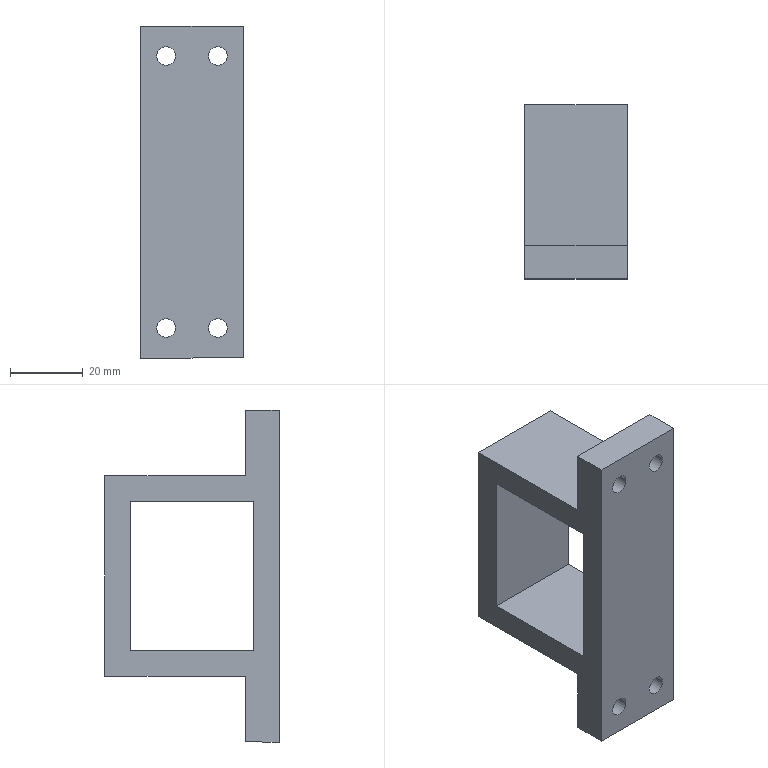Component | SolidWorks | EndCap-2 | 1 solid | 22 faces | box 28 x 47.79 x 91 mm | volume 43383 mm3 | plane 14 | cylinder 8 | commonest cylinder face diameters 5.084 x8
STEP:
#1=CARTESIAN_POINT('',(6.308,1.43,1.468));
#2=VERTEX_POINT('',#1);
#3=CARTESIAN_POINT('',(6.108,1.43,1.468));
#4=VERTEX_POINT('',#3);
#5=CARTESIAN_POINT('',(6.208,1.43,1.468));
#6=DIRECTION('',(0.,-1.,-0.));
#7=DIRECTION('',(0.,0.,-1.));
#8=AXIS2_PLACEMENT_3D('',#5,#6,#7);
#9=CIRCLE('',#8,0.1001);
#10=EDGE_CURVE('',#2,#4,#9,.T.);
#11=ORIENTED_EDGE('',*,*,#10,.T.);
#12=CARTESIAN_POINT('',(6.108,1.794,1.468));
#13=VERTEX_POINT('',#12);
#14=CARTESIAN_POINT('',(6.108,1.263,1.468));
#15=DIRECTION('',(-0.,1.,0.));
#16=VECTOR('',#15,39.37);
#17=LINE('',#14,#16);
#18=EDGE_CURVE('',#4,#13,#17,.T.);
#19=ORIENTED_EDGE('',*,*,#18,.T.);
#20=CARTESIAN_POINT('',(6.308,1.794,1.468));
#21=VERTEX_POINT('',#20);
#22=CARTESIAN_POINT('',(6.208,1.794,1.468));
#23=DIRECTION('',(-0.,1.,0.));
#24=DIRECTION('',(-1.,0.,0.));
#25=AXIS2_PLACEMENT_3D('',#22,#23,#24);
#26=CIRCLE('',#25,0.1001);
#27=EDGE_CURVE('',#13,#21,#26,.T.);
#28=ORIENTED_EDGE('',*,*,#27,.T.);
#29=CARTESIAN_POINT('',(6.308,1.263,1.468));
#30=DIRECTION('',(-0.,1.,0.));
#31=VECTOR('',#30,39.37);
#32=LINE('',#29,#31);
#33=EDGE_CURVE('',#2,#21,#32,.T.);
#34=ORIENTED_EDGE('',*,*,#33,.F.);
#35=EDGE_LOOP('',(#11,#19,#28,#34));
#36=FACE_OUTER_BOUND('',#35,.T.);
#37=CARTESIAN_POINT('',(6.208,1.263,1.468));
#38=DIRECTION('',(-0.,1.,0.));
#39=DIRECTION('',(1.,0.,0.));
#40=AXIS2_PLACEMENT_3D('',#37,#38,#39);
#41=CYLINDRICAL_SURFACE('',#40,0.1001);
#42=ADVANCED_FACE('',(#36),#41,.F.);
#43=CARTESIAN_POINT('',(6.867,1.43,1.468));
#44=VERTEX_POINT('',#43);
#45=CARTESIAN_POINT('',(6.667,1.43,1.468));
#46=VERTEX_POINT('',#45);
#47=CARTESIAN_POINT('',(6.767,1.43,1.468));
#48=DIRECTION('',(0.,-1.,-0.));
#49=DIRECTION('',(0.,0.,-1.));
#50=AXIS2_PLACEMENT_3D('',#47,#48,#49);
#51=CIRCLE('',#50,0.1001);
#52=EDGE_CURVE('',#44,#46,#51,.T.);
#53=ORIENTED_EDGE('',*,*,#52,.T.);
#54=CARTESIAN_POINT('',(6.667,1.794,1.468));
#55=VERTEX_POINT('',#54);
#56=CARTESIAN_POINT('',(6.667,1.263,1.468));
#57=DIRECTION('',(-0.,1.,0.));
#58=VECTOR('',#57,39.37);
#59=LINE('',#56,#58);
#60=EDGE_CURVE('',#46,#55,#59,.T.);
#61=ORIENTED_EDGE('',*,*,#60,.T.);
#62=CARTESIAN_POINT('',(6.867,1.794,1.468));
#63=VERTEX_POINT('',#62);
#64=CARTESIAN_POINT('',(6.767,1.794,1.468));
#65=DIRECTION('',(-0.,1.,0.));
#66=DIRECTION('',(1.,0.,0.));
#67=AXIS2_PLACEMENT_3D('',#64,#65,#66);
#68=CIRCLE('',#67,0.1001);
#69=EDGE_CURVE('',#55,#63,#68,.T.);
#70=ORIENTED_EDGE('',*,*,#69,.T.);
#71=CARTESIAN_POINT('',(6.867,1.263,1.468));
#72=DIRECTION('',(-0.,1.,0.));
#73=VECTOR('',#72,39.37);
#74=LINE('',#71,#73);
#75=EDGE_CURVE('',#44,#63,#74,.T.);
#76=ORIENTED_EDGE('',*,*,#75,.F.);
#77=EDGE_LOOP('',(#53,#61,#70,#76));
#78=FACE_OUTER_BOUND('',#77,.T.);
#79=CARTESIAN_POINT('',(6.767,1.263,1.468));
#80=DIRECTION('',(-0.,1.,0.));
#81=DIRECTION('',(1.,0.,0.));
#82=AXIS2_PLACEMENT_3D('',#79,#80,#81);
#83=CYLINDRICAL_SURFACE('',#82,0.1001);
#84=ADVANCED_FACE('',(#78),#83,.F.);
#85=CARTESIAN_POINT('',(6.867,1.43,-1.468));
#86=VERTEX_POINT('',#85);
#87=CARTESIAN_POINT('',(6.667,1.43,-1.468));
#88=VERTEX_POINT('',#87);
#89=CARTESIAN_POINT('',(6.767,1.43,-1.468));
#90=DIRECTION('',(0.,-1.,-0.));
#91=DIRECTION('',(0.,0.,-1.));
#92=AXIS2_PLACEMENT_3D('',#89,#90,#91);
#93=CIRCLE('',#92,0.1001);
#94=EDGE_CURVE('',#86,#88,#93,.T.);
#95=ORIENTED_EDGE('',*,*,#94,.T.);
#96=CARTESIAN_POINT('',(6.667,1.794,-1.468));
#97=VERTEX_POINT('',#96);
#98=CARTESIAN_POINT('',(6.667,1.263,-1.468));
#99=DIRECTION('',(-0.,1.,0.));
#100=VECTOR('',#99,39.37);
#101=LINE('',#98,#100);
#102=EDGE_CURVE('',#88,#97,#101,.T.);
#103=ORIENTED_EDGE('',*,*,#102,.T.);
#104=CARTESIAN_POINT('',(6.867,1.794,-1.468));
#105=VERTEX_POINT('',#104);
#106=CARTESIAN_POINT('',(6.767,1.794,-1.468));
#107=DIRECTION('',(-0.,1.,0.));
#108=DIRECTION('',(-1.,0.,0.));
#109=AXIS2_PLACEMENT_3D('',#106,#107,#108);
#110=CIRCLE('',#109,0.1001);
#111=EDGE_CURVE('',#97,#105,#110,.T.);
#112=ORIENTED_EDGE('',*,*,#111,.T.);
#113=CARTESIAN_POINT('',(6.867,1.263,-1.468));
#114=DIRECTION('',(-0.,1.,0.));
#115=VECTOR('',#114,39.37);
#116=LINE('',#113,#115);
#117=EDGE_CURVE('',#86,#105,#116,.T.);
#118=ORIENTED_EDGE('',*,*,#117,.F.);
#119=EDGE_LOOP('',(#95,#103,#112,#118));
#120=FACE_OUTER_BOUND('',#119,.T.);
#121=CARTESIAN_POINT('',(6.767,1.263,-1.468));
#122=DIRECTION('',(-0.,1.,0.));
#123=DIRECTION('',(1.,0.,0.));
#124=AXIS2_PLACEMENT_3D('',#121,#122,#123);
#125=CYLINDRICAL_SURFACE('',#124,0.1001);
#126=ADVANCED_FACE('',(#120),#125,.F.);
#127=CARTESIAN_POINT('',(6.308,1.43,-1.468));
#128=VERTEX_POINT('',#127);
#129=CARTESIAN_POINT('',(6.108,1.43,-1.468));
#130=VERTEX_POINT('',#129);
#131=CARTESIAN_POINT('',(6.208,1.43,-1.468));
#132=DIRECTION('',(0.,-1.,-0.));
#133=DIRECTION('',(0.,0.,-1.));
#134=AXIS2_PLACEMENT_3D('',#131,#132,#133);
#135=CIRCLE('',#134,0.1001);
#136=EDGE_CURVE('',#128,#130,#135,.T.);
#137=ORIENTED_EDGE('',*,*,#136,.T.);
#138=CARTESIAN_POINT('',(6.108,1.794,-1.468));
#139=VERTEX_POINT('',#138);
#140=CARTESIAN_POINT('',(6.108,1.263,-1.468));
#141=DIRECTION('',(-0.,1.,0.));
#142=VECTOR('',#141,39.37);
#143=LINE('',#140,#142);
#144=EDGE_CURVE('',#130,#139,#143,.T.);
#145=ORIENTED_EDGE('',*,*,#144,.T.);
#146=CARTESIAN_POINT('',(6.308,1.794,-1.468));
#147=VERTEX_POINT('',#146);
#148=CARTESIAN_POINT('',(6.208,1.794,-1.468));
#149=DIRECTION('',(-0.,1.,0.));
#150=DIRECTION('',(1.,0.,0.));
#151=AXIS2_PLACEMENT_3D('',#148,#149,#150);
#152=CIRCLE('',#151,0.1001);
#153=EDGE_CURVE('',#139,#147,#152,.T.);
#154=ORIENTED_EDGE('',*,*,#153,.T.);
#155=CARTESIAN_POINT('',(6.308,1.263,-1.468));
#156=DIRECTION('',(-0.,1.,0.));
#157=VECTOR('',#156,39.37);
#158=LINE('',#155,#157);
#159=EDGE_CURVE('',#128,#147,#158,.T.);
#160=ORIENTED_EDGE('',*,*,#159,.F.);
#161=EDGE_LOOP('',(#137,#145,#154,#160));
#162=FACE_OUTER_BOUND('',#161,.T.);
#163=CARTESIAN_POINT('',(6.208,1.263,-1.468));
#164=DIRECTION('',(-0.,1.,0.));
#165=DIRECTION('',(1.,0.,0.));
#166=AXIS2_PLACEMENT_3D('',#163,#164,#165);
#167=CYLINDRICAL_SURFACE('',#166,0.1001);
#168=ADVANCED_FACE('',(#162),#167,.F.);
#169=CARTESIAN_POINT('',(5.936,3.312,1.083));
#170=VERTEX_POINT('',#169);
#171=CARTESIAN_POINT('',(7.039,3.312,1.083));
#172=VERTEX_POINT('',#171);
#173=CARTESIAN_POINT('',(6.251,3.312,1.083));
#174=DIRECTION('',(1.,0.,0.));
#175=VECTOR('',#174,39.37);
#176=LINE('',#173,#175);
#177=EDGE_CURVE('',#170,#172,#176,.T.);
#178=ORIENTED_EDGE('',*,*,#177,.F.);
#179=CARTESIAN_POINT('',(5.936,1.794,1.083));
#180=VERTEX_POINT('',#179);
#181=CARTESIAN_POINT('',(5.936,1.794,1.083));
#182=DIRECTION('',(0.,-1.,-0.));
#183=VECTOR('',#182,39.37);
#184=LINE('',#181,#183);
#185=EDGE_CURVE('',#170,#180,#184,.T.);
#186=ORIENTED_EDGE('',*,*,#185,.T.);
#187=CARTESIAN_POINT('',(7.039,1.794,1.083));
#188=VERTEX_POINT('',#187);
#189=CARTESIAN_POINT('',(-3.832,1.794,1.083));
#190=DIRECTION('',(1.,0.,0.));
#191=VECTOR('',#190,39.37);
#192=LINE('',#189,#191);
#193=EDGE_CURVE('',#180,#188,#192,.T.);
#194=ORIENTED_EDGE('',*,*,#193,.T.);
#195=CARTESIAN_POINT('',(7.039,3.312,1.083));
#196=DIRECTION('',(0.,-1.,-0.));
#197=VECTOR('',#196,39.37);
#198=LINE('',#195,#197);
#199=EDGE_CURVE('',#172,#188,#198,.T.);
#200=ORIENTED_EDGE('',*,*,#199,.F.);
#201=EDGE_LOOP('',(#178,#186,#194,#200));
#202=FACE_OUTER_BOUND('',#201,.T.);
#203=CARTESIAN_POINT('',(6.251,3.312,1.083));
#204=DIRECTION('',(-0.,-0.,1.));
#205=DIRECTION('',(0.,-1.,-0.));
#206=AXIS2_PLACEMENT_3D('',#203,#204,#205);
#207=PLANE('',#206);
#208=ADVANCED_FACE('',(#202),#207,.T.);
#209=CARTESIAN_POINT('',(7.039,3.312,-1.083));
#210=VERTEX_POINT('',#209);
#211=CARTESIAN_POINT('',(7.039,3.312,-1.083));
#212=DIRECTION('',(-0.,-0.,1.));
#213=VECTOR('',#212,39.37);
#214=LINE('',#211,#213);
#215=EDGE_CURVE('',#210,#172,#214,.T.);
#216=ORIENTED_EDGE('',*,*,#215,.F.);
#217=CARTESIAN_POINT('',(5.936,3.312,-1.083));
#218=VERTEX_POINT('',#217);
#219=CARTESIAN_POINT('',(6.251,3.312,-1.083));
#220=DIRECTION('',(1.,0.,0.));
#221=VECTOR('',#220,39.37);
#222=LINE('',#219,#221);
#223=EDGE_CURVE('',#218,#210,#222,.T.);
#224=ORIENTED_EDGE('',*,*,#223,.F.);
#225=CARTESIAN_POINT('',(5.936,3.312,1.083));
#226=DIRECTION('',(-0.,-0.,1.));
#227=VECTOR('',#226,39.37);
#228=LINE('',#225,#227);
#229=EDGE_CURVE('',#218,#170,#228,.T.);
#230=ORIENTED_EDGE('',*,*,#229,.T.);
#231=ORIENTED_EDGE('',*,*,#177,.T.);
#232=EDGE_LOOP('',(#216,#224,#230,#231));
#233=FACE_OUTER_BOUND('',#232,.T.);
#234=CARTESIAN_POINT('',(6.251,3.312,-1.083));
#235=DIRECTION('',(-0.,1.,0.));
#236=DIRECTION('',(-0.,-0.,1.));
#237=AXIS2_PLACEMENT_3D('',#234,#235,#236);
#238=PLANE('',#237);
#239=ADVANCED_FACE('',(#233),#238,.T.);
#240=CARTESIAN_POINT('',(5.936,1.794,-1.083));
#241=VERTEX_POINT('',#240);
#242=CARTESIAN_POINT('',(7.039,1.794,-1.083));
#243=VERTEX_POINT('',#242);
#244=CARTESIAN_POINT('',(-3.832,1.794,-1.083));
#245=DIRECTION('',(1.,0.,0.));
#246=VECTOR('',#245,39.37);
#247=LINE('',#244,#246);
#248=EDGE_CURVE('',#241,#243,#247,.T.);
#249=ORIENTED_EDGE('',*,*,#248,.F.);
#250=CARTESIAN_POINT('',(5.936,3.312,-1.083));
#251=DIRECTION('',(-0.,1.,0.));
#252=VECTOR('',#251,39.37);
#253=LINE('',#250,#252);
#254=EDGE_CURVE('',#241,#218,#253,.T.);
#255=ORIENTED_EDGE('',*,*,#254,.T.);
#256=ORIENTED_EDGE('',*,*,#223,.T.);
#257=CARTESIAN_POINT('',(7.039,1.43,-1.083));
#258=DIRECTION('',(-0.,1.,0.));
#259=VECTOR('',#258,39.37);
#260=LINE('',#257,#259);
#261=EDGE_CURVE('',#243,#210,#260,.T.);
#262=ORIENTED_EDGE('',*,*,#261,.F.);
#263=EDGE_LOOP('',(#249,#255,#256,#262));
#264=FACE_OUTER_BOUND('',#263,.T.);
#265=CARTESIAN_POINT('',(6.251,1.43,-1.083));
#266=DIRECTION('',(0.,0.,-1.));
#267=DIRECTION('',(-0.,1.,0.));
#268=AXIS2_PLACEMENT_3D('',#265,#266,#267);
#269=PLANE('',#268);
#270=ADVANCED_FACE('',(#264),#269,.T.);
#271=ORIENTED_EDGE('',*,*,#94,.F.);
#272=CARTESIAN_POINT('',(6.767,1.43,-1.468));
#273=DIRECTION('',(0.,-1.,-0.));
#274=DIRECTION('',(0.,0.,-1.));
#275=AXIS2_PLACEMENT_3D('',#272,#273,#274);
#276=CIRCLE('',#275,0.1001);
#277=EDGE_CURVE('',#88,#86,#276,.T.);
#278=ORIENTED_EDGE('',*,*,#277,.F.);
#279=EDGE_LOOP('',(#271,#278));
#280=FACE_BOUND('',#279,.T.);
#281=ORIENTED_EDGE('',*,*,#10,.F.);
#282=CARTESIAN_POINT('',(6.208,1.43,1.468));
#283=DIRECTION('',(0.,-1.,-0.));
#284=DIRECTION('',(0.,0.,-1.));
#285=AXIS2_PLACEMENT_3D('',#282,#283,#284);
#286=CIRCLE('',#285,0.1001);
#287=EDGE_CURVE('',#4,#2,#286,.T.);
#288=ORIENTED_EDGE('',*,*,#287,.F.);
#289=EDGE_LOOP('',(#281,#288));
#290=FACE_BOUND('',#289,.T.);
#291=ORIENTED_EDGE('',*,*,#52,.F.);
#292=CARTESIAN_POINT('',(6.767,1.43,1.468));
#293=DIRECTION('',(0.,-1.,-0.));
#294=DIRECTION('',(0.,0.,-1.));
#295=AXIS2_PLACEMENT_3D('',#292,#293,#294);
#296=CIRCLE('',#295,0.1001);
#297=EDGE_CURVE('',#46,#44,#296,.T.);
#298=ORIENTED_EDGE('',*,*,#297,.F.);
#299=EDGE_LOOP('',(#291,#298));
#300=FACE_BOUND('',#299,.T.);
#301=ORIENTED_EDGE('',*,*,#136,.F.);
#302=CARTESIAN_POINT('',(6.208,1.43,-1.468));
#303=DIRECTION('',(0.,-1.,-0.));
#304=DIRECTION('',(0.,0.,-1.));
#305=AXIS2_PLACEMENT_3D('',#302,#303,#304);
#306=CIRCLE('',#305,0.1001);
#307=EDGE_CURVE('',#130,#128,#306,.T.);
#308=ORIENTED_EDGE('',*,*,#307,.F.);
#309=EDGE_LOOP('',(#301,#308));
#310=FACE_BOUND('',#309,.T.);
#311=CARTESIAN_POINT('',(7.039,1.43,1.791));
#312=VERTEX_POINT('',#311);
#313=CARTESIAN_POINT('',(7.039,1.43,-1.791));
#314=VERTEX_POINT('',#313);
#315=CARTESIAN_POINT('',(7.039,1.43,1.083));
#316=DIRECTION('',(0.,0.,-1.));
#317=VECTOR('',#316,39.37);
#318=LINE('',#315,#317);
#319=EDGE_CURVE('',#312,#314,#318,.T.);
#320=ORIENTED_EDGE('',*,*,#319,.F.);
#321=CARTESIAN_POINT('',(5.936,1.43,1.791));
#322=VERTEX_POINT('',#321);
#323=CARTESIAN_POINT('',(-3.832,1.43,1.791));
#324=DIRECTION('',(1.,0.,0.));
#325=VECTOR('',#324,39.37);
#326=LINE('',#323,#325);
#327=EDGE_CURVE('',#322,#312,#326,.T.);
#328=ORIENTED_EDGE('',*,*,#327,.F.);
#329=CARTESIAN_POINT('',(5.936,1.43,-1.791));
#330=VERTEX_POINT('',#329);
#331=CARTESIAN_POINT('',(5.936,1.43,-1.791));
#332=DIRECTION('',(0.,0.,-1.));
#333=VECTOR('',#332,39.37);
#334=LINE('',#331,#333);
#335=EDGE_CURVE('',#322,#330,#334,.T.);
#336=ORIENTED_EDGE('',*,*,#335,.T.);
#337=CARTESIAN_POINT('',(-3.832,1.43,-1.791));
#338=DIRECTION('',(1.,0.,0.));
#339=VECTOR('',#338,39.37);
#340=LINE('',#337,#339);
#341=EDGE_CURVE('',#330,#314,#340,.T.);
#342=ORIENTED_EDGE('',*,*,#341,.T.);
#343=EDGE_LOOP('',(#320,#328,#336,#342));
#344=FACE_OUTER_BOUND('',#343,.T.);
#345=CARTESIAN_POINT('',(6.251,1.43,1.083));
#346=DIRECTION('',(0.,-1.,-0.));
#347=DIRECTION('',(0.,0.,-1.));
#348=AXIS2_PLACEMENT_3D('',#345,#346,#347);
#349=PLANE('',#348);
#350=ADVANCED_FACE('',(#280,#290,#300,#310,#344),#349,.T.);
#351=CARTESIAN_POINT('',(7.039,1.706,-0.8071));
#352=VERTEX_POINT('',#351);
#353=CARTESIAN_POINT('',(7.039,3.036,-0.8071));
#354=VERTEX_POINT('',#353);
#355=CARTESIAN_POINT('',(7.039,1.706,-0.8071));
#356=DIRECTION('',(-0.,1.,0.));
#357=VECTOR('',#356,39.37);
#358=LINE('',#355,#357);
#359=EDGE_CURVE('',#352,#354,#358,.T.);
#360=ORIENTED_EDGE('',*,*,#359,.F.);
#361=CARTESIAN_POINT('',(7.039,1.706,0.8071));
#362=VERTEX_POINT('',#361);
#363=CARTESIAN_POINT('',(7.039,1.706,0.8071));
#364=DIRECTION('',(0.,0.,-1.));
#365=VECTOR('',#364,39.37);
#366=LINE('',#363,#365);
#367=EDGE_CURVE('',#362,#352,#366,.T.);
#368=ORIENTED_EDGE('',*,*,#367,.F.);
#369=CARTESIAN_POINT('',(7.039,3.036,0.8071));
#370=VERTEX_POINT('',#369);
#371=CARTESIAN_POINT('',(7.039,3.036,0.8071));
#372=DIRECTION('',(0.,-1.,-0.));
#373=VECTOR('',#372,39.37);
#374=LINE('',#371,#373);
#375=EDGE_CURVE('',#370,#362,#374,.T.);
#376=ORIENTED_EDGE('',*,*,#375,.F.);
#377=CARTESIAN_POINT('',(7.039,3.036,-0.8071));
#378=DIRECTION('',(-0.,-0.,1.));
#379=VECTOR('',#378,39.37);
#380=LINE('',#377,#379);
#381=EDGE_CURVE('',#354,#370,#380,.T.);
#382=ORIENTED_EDGE('',*,*,#381,.F.);
#383=EDGE_LOOP('',(#360,#368,#376,#382));
#384=FACE_BOUND('',#383,.T.);
#385=ORIENTED_EDGE('',*,*,#199,.T.);
#386=CARTESIAN_POINT('',(7.039,1.794,1.791));
#387=VERTEX_POINT('',#386);
#388=CARTESIAN_POINT('',(7.039,1.794,1.791));
#389=DIRECTION('',(0.,0.,-1.));
#390=VECTOR('',#389,39.37);
#391=LINE('',#388,#390);
#392=EDGE_CURVE('',#387,#188,#391,.T.);
#393=ORIENTED_EDGE('',*,*,#392,.F.);
#394=CARTESIAN_POINT('',(7.039,3.036,1.791));
#395=DIRECTION('',(-0.,1.,0.));
#396=VECTOR('',#395,39.37);
#397=LINE('',#394,#396);
#398=EDGE_CURVE('',#312,#387,#397,.T.);
#399=ORIENTED_EDGE('',*,*,#398,.F.);
#400=ORIENTED_EDGE('',*,*,#319,.T.);
#401=CARTESIAN_POINT('',(7.039,1.794,-1.791));
#402=VERTEX_POINT('',#401);
#403=CARTESIAN_POINT('',(7.039,3.036,-1.791));
#404=DIRECTION('',(-0.,1.,0.));
#405=VECTOR('',#404,39.37);
#406=LINE('',#403,#405);
#407=EDGE_CURVE('',#314,#402,#406,.T.);
#408=ORIENTED_EDGE('',*,*,#407,.T.);
#409=CARTESIAN_POINT('',(7.039,1.794,-1.791));
#410=DIRECTION('',(-0.,-0.,1.));
#411=VECTOR('',#410,39.37);
#412=LINE('',#409,#411);
#413=EDGE_CURVE('',#402,#243,#412,.T.);
#414=ORIENTED_EDGE('',*,*,#413,.T.);
#415=ORIENTED_EDGE('',*,*,#261,.T.);
#416=ORIENTED_EDGE('',*,*,#215,.T.);
#417=EDGE_LOOP('',(#385,#393,#399,#400,#408,#414,#415,#416));
#418=FACE_OUTER_BOUND('',#417,.T.);
#419=CARTESIAN_POINT('',(7.039,3.036,-0.));
#420=DIRECTION('',(1.,0.,0.));
#421=DIRECTION('',(0.,-1.,-0.));
#422=AXIS2_PLACEMENT_3D('',#419,#420,#421);
#423=PLANE('',#422);
#424=ADVANCED_FACE('',(#384,#418),#423,.T.);
#425=ORIENTED_EDGE('',*,*,#359,.T.);
#426=CARTESIAN_POINT('',(5.936,3.036,-0.8071));
#427=VERTEX_POINT('',#426);
#428=CARTESIAN_POINT('',(6.251,3.036,-0.8071));
#429=DIRECTION('',(1.,0.,0.));
#430=VECTOR('',#429,39.37);
#431=LINE('',#428,#430);
#432=EDGE_CURVE('',#427,#354,#431,.T.);
#433=ORIENTED_EDGE('',*,*,#432,.F.);
#434=CARTESIAN_POINT('',(5.936,1.706,-0.8071));
#435=VERTEX_POINT('',#434);
#436=CARTESIAN_POINT('',(5.936,1.706,-0.8071));
#437=DIRECTION('',(-0.,1.,0.));
#438=VECTOR('',#437,39.37);
#439=LINE('',#436,#438);
#440=EDGE_CURVE('',#435,#427,#439,.T.);
#441=ORIENTED_EDGE('',*,*,#440,.F.);
#442=CARTESIAN_POINT('',(6.251,1.706,-0.8071));
#443=DIRECTION('',(1.,0.,0.));
#444=VECTOR('',#443,39.37);
#445=LINE('',#442,#444);
#446=EDGE_CURVE('',#435,#352,#445,.T.);
#447=ORIENTED_EDGE('',*,*,#446,.T.);
#448=EDGE_LOOP('',(#425,#433,#441,#447));
#449=FACE_OUTER_BOUND('',#448,.T.);
#450=CARTESIAN_POINT('',(6.251,1.706,-0.8071));
#451=DIRECTION('',(0.,0.,-1.));
#452=DIRECTION('',(-0.,1.,0.));
#453=AXIS2_PLACEMENT_3D('',#450,#451,#452);
#454=PLANE('',#453);
#455=ADVANCED_FACE('',(#449),#454,.F.);
#456=ORIENTED_EDGE('',*,*,#367,.T.);
#457=ORIENTED_EDGE('',*,*,#446,.F.);
#458=CARTESIAN_POINT('',(5.936,1.706,0.8071));
#459=VERTEX_POINT('',#458);
#460=CARTESIAN_POINT('',(5.936,1.706,0.8071));
#461=DIRECTION('',(0.,0.,-1.));
#462=VECTOR('',#461,39.37);
#463=LINE('',#460,#462);
#464=EDGE_CURVE('',#459,#435,#463,.T.);
#465=ORIENTED_EDGE('',*,*,#464,.F.);
#466=CARTESIAN_POINT('',(6.251,1.706,0.8071));
#467=DIRECTION('',(1.,0.,0.));
#468=VECTOR('',#467,39.37);
#469=LINE('',#466,#468);
#470=EDGE_CURVE('',#459,#362,#469,.T.);
#471=ORIENTED_EDGE('',*,*,#470,.T.);
#472=EDGE_LOOP('',(#456,#457,#465,#471));
#473=FACE_OUTER_BOUND('',#472,.T.);
#474=CARTESIAN_POINT('',(6.251,1.706,0.8071));
#475=DIRECTION('',(0.,-1.,-0.));
#476=DIRECTION('',(0.,0.,-1.));
#477=AXIS2_PLACEMENT_3D('',#474,#475,#476);
#478=PLANE('',#477);
#479=ADVANCED_FACE('',(#473),#478,.F.);
#480=ORIENTED_EDGE('',*,*,#375,.T.);
#481=ORIENTED_EDGE('',*,*,#470,.F.);
#482=CARTESIAN_POINT('',(5.936,3.036,0.8071));
#483=VERTEX_POINT('',#482);
#484=CARTESIAN_POINT('',(5.936,3.036,0.8071));
#485=DIRECTION('',(0.,-1.,-0.));
#486=VECTOR('',#485,39.37);
#487=LINE('',#484,#486);
#488=EDGE_CURVE('',#483,#459,#487,.T.);
#489=ORIENTED_EDGE('',*,*,#488,.F.);
#490=CARTESIAN_POINT('',(6.251,3.036,0.8071));
#491=DIRECTION('',(1.,0.,0.));
#492=VECTOR('',#491,39.37);
#493=LINE('',#490,#492);
#494=EDGE_CURVE('',#483,#370,#493,.T.);
#495=ORIENTED_EDGE('',*,*,#494,.T.);
#496=EDGE_LOOP('',(#480,#481,#489,#495));
#497=FACE_OUTER_BOUND('',#496,.T.);
#498=CARTESIAN_POINT('',(6.251,3.036,0.8071));
#499=DIRECTION('',(-0.,-0.,1.));
#500=DIRECTION('',(0.,-1.,-0.));
#501=AXIS2_PLACEMENT_3D('',#498,#499,#500);
#502=PLANE('',#501);
#503=ADVANCED_FACE('',(#497),#502,.F.);
#504=ORIENTED_EDGE('',*,*,#381,.T.);
#505=ORIENTED_EDGE('',*,*,#494,.F.);
#506=CARTESIAN_POINT('',(5.936,3.036,-0.8071));
#507=DIRECTION('',(-0.,-0.,1.));
#508=VECTOR('',#507,39.37);
#509=LINE('',#506,#508);
#510=EDGE_CURVE('',#427,#483,#509,.T.);
#511=ORIENTED_EDGE('',*,*,#510,.F.);
#512=ORIENTED_EDGE('',*,*,#432,.T.);
#513=EDGE_LOOP('',(#504,#505,#511,#512));
#514=FACE_OUTER_BOUND('',#513,.T.);
#515=CARTESIAN_POINT('',(6.251,3.036,-0.8071));
#516=DIRECTION('',(-0.,1.,0.));
#517=DIRECTION('',(-0.,-0.,1.));
#518=AXIS2_PLACEMENT_3D('',#515,#516,#517);
#519=PLANE('',#518);
#520=ADVANCED_FACE('',(#514),#519,.F.);
#521=CARTESIAN_POINT('',(6.208,1.794,1.468));
#522=DIRECTION('',(-0.,1.,0.));
#523=DIRECTION('',(-1.,0.,0.));
#524=AXIS2_PLACEMENT_3D('',#521,#522,#523);
#525=CIRCLE('',#524,0.1001);
#526=EDGE_CURVE('',#21,#13,#525,.T.);
#527=ORIENTED_EDGE('',*,*,#526,.F.);
#528=ORIENTED_EDGE('',*,*,#27,.F.);
#529=EDGE_LOOP('',(#527,#528));
#530=FACE_BOUND('',#529,.T.);
#531=CARTESIAN_POINT('',(6.767,1.794,1.468));
#532=DIRECTION('',(-0.,1.,0.));
#533=DIRECTION('',(1.,0.,0.));
#534=AXIS2_PLACEMENT_3D('',#531,#532,#533);
#535=CIRCLE('',#534,0.1001);
#536=EDGE_CURVE('',#63,#55,#535,.T.);
#537=ORIENTED_EDGE('',*,*,#536,.F.);
#538=ORIENTED_EDGE('',*,*,#69,.F.);
#539=EDGE_LOOP('',(#537,#538));
#540=FACE_BOUND('',#539,.T.);
#541=ORIENTED_EDGE('',*,*,#193,.F.);
#542=CARTESIAN_POINT('',(5.936,1.794,1.791));
#543=VERTEX_POINT('',#542);
#544=CARTESIAN_POINT('',(5.936,1.794,1.791));
#545=DIRECTION('',(-0.,-0.,1.));
#546=VECTOR('',#545,39.37);
#547=LINE('',#544,#546);
#548=EDGE_CURVE('',#180,#543,#547,.T.);
#549=ORIENTED_EDGE('',*,*,#548,.T.);
#550=CARTESIAN_POINT('',(-3.832,1.794,1.791));
#551=DIRECTION('',(1.,0.,0.));
#552=VECTOR('',#551,39.37);
#553=LINE('',#550,#552);
#554=EDGE_CURVE('',#543,#387,#553,.T.);
#555=ORIENTED_EDGE('',*,*,#554,.T.);
#556=ORIENTED_EDGE('',*,*,#392,.T.);
#557=EDGE_LOOP('',(#541,#549,#555,#556));
#558=FACE_OUTER_BOUND('',#557,.T.);
#559=CARTESIAN_POINT('',(-3.832,1.794,1.791));
#560=DIRECTION('',(-0.,1.,0.));
#561=DIRECTION('',(-0.,-0.,1.));
#562=AXIS2_PLACEMENT_3D('',#559,#560,#561);
#563=PLANE('',#562);
#564=ADVANCED_FACE('',(#530,#540,#558),#563,.T.);
#565=ORIENTED_EDGE('',*,*,#554,.F.);
#566=CARTESIAN_POINT('',(5.936,1.43,1.791));
#567=DIRECTION('',(0.,-1.,0.));
#568=VECTOR('',#567,39.37);
#569=LINE('',#566,#568);
#570=EDGE_CURVE('',#543,#322,#569,.T.);
#571=ORIENTED_EDGE('',*,*,#570,.T.);
#572=ORIENTED_EDGE('',*,*,#327,.T.);
#573=ORIENTED_EDGE('',*,*,#398,.T.);
#574=EDGE_LOOP('',(#565,#571,#572,#573));
#575=FACE_OUTER_BOUND('',#574,.T.);
#576=CARTESIAN_POINT('',(-3.832,3.036,1.791));
#577=DIRECTION('',(-0.,-0.,1.));
#578=DIRECTION('',(0.,-1.,-0.));
#579=AXIS2_PLACEMENT_3D('',#576,#577,#578);
#580=PLANE('',#579);
#581=ADVANCED_FACE('',(#575),#580,.T.);
#582=CARTESIAN_POINT('',(6.767,1.794,-1.468));
#583=DIRECTION('',(-0.,1.,0.));
#584=DIRECTION('',(-1.,0.,0.));
#585=AXIS2_PLACEMENT_3D('',#582,#583,#584);
#586=CIRCLE('',#585,0.1001);
#587=EDGE_CURVE('',#105,#97,#586,.T.);
#588=ORIENTED_EDGE('',*,*,#587,.F.);
#589=ORIENTED_EDGE('',*,*,#111,.F.);
#590=EDGE_LOOP('',(#588,#589));
#591=FACE_BOUND('',#590,.T.);
#592=CARTESIAN_POINT('',(6.208,1.794,-1.468));
#593=DIRECTION('',(-0.,1.,0.));
#594=DIRECTION('',(1.,0.,0.));
#595=AXIS2_PLACEMENT_3D('',#592,#593,#594);
#596=CIRCLE('',#595,0.1001);
#597=EDGE_CURVE('',#147,#139,#596,.T.);
#598=ORIENTED_EDGE('',*,*,#597,.F.);
#599=ORIENTED_EDGE('',*,*,#153,.F.);
#600=EDGE_LOOP('',(#598,#599));
#601=FACE_BOUND('',#600,.T.);
#602=ORIENTED_EDGE('',*,*,#248,.T.);
#603=ORIENTED_EDGE('',*,*,#413,.F.);
#604=CARTESIAN_POINT('',(5.936,1.794,-1.791));
#605=VERTEX_POINT('',#604);
#606=CARTESIAN_POINT('',(-3.832,1.794,-1.791));
#607=DIRECTION('',(1.,0.,0.));
#608=VECTOR('',#607,39.37);
#609=LINE('',#606,#608);
#610=EDGE_CURVE('',#605,#402,#609,.T.);
#611=ORIENTED_EDGE('',*,*,#610,.F.);
#612=CARTESIAN_POINT('',(5.936,1.794,-1.083));
#613=DIRECTION('',(-0.,-0.,1.));
#614=VECTOR('',#613,39.37);
#615=LINE('',#612,#614);
#616=EDGE_CURVE('',#605,#241,#615,.T.);
#617=ORIENTED_EDGE('',*,*,#616,.T.);
#618=EDGE_LOOP('',(#602,#603,#611,#617));
#619=FACE_OUTER_BOUND('',#618,.T.);
#620=CARTESIAN_POINT('',(-3.832,1.794,-1.791));
#621=DIRECTION('',(0.,-1.,-0.));
#622=DIRECTION('',(0.,0.,-1.));
#623=AXIS2_PLACEMENT_3D('',#620,#621,#622);
#624=PLANE('',#623);
#625=ADVANCED_FACE('',(#591,#601,#619),#624,.F.);
#626=ORIENTED_EDGE('',*,*,#610,.T.);
#627=ORIENTED_EDGE('',*,*,#407,.F.);
#628=ORIENTED_EDGE('',*,*,#341,.F.);
#629=CARTESIAN_POINT('',(5.936,1.794,-1.791));
#630=DIRECTION('',(-0.,1.,0.));
#631=VECTOR('',#630,39.37);
#632=LINE('',#629,#631);
#633=EDGE_CURVE('',#330,#605,#632,.T.);
#634=ORIENTED_EDGE('',*,*,#633,.T.);
#635=EDGE_LOOP('',(#626,#627,#628,#634));
#636=FACE_OUTER_BOUND('',#635,.T.);
#637=CARTESIAN_POINT('',(-3.832,3.036,-1.791));
#638=DIRECTION('',(0.,0.,-1.));
#639=DIRECTION('',(0.,-1.,-0.));
#640=AXIS2_PLACEMENT_3D('',#637,#638,#639);
#641=PLANE('',#640);
#642=ADVANCED_FACE('',(#636),#641,.T.);
#643=ORIENTED_EDGE('',*,*,#464,.T.);
#644=ORIENTED_EDGE('',*,*,#440,.T.);
#645=ORIENTED_EDGE('',*,*,#510,.T.);
#646=ORIENTED_EDGE('',*,*,#488,.T.);
#647=EDGE_LOOP('',(#643,#644,#645,#646));
#648=FACE_BOUND('',#647,.T.);
#649=ORIENTED_EDGE('',*,*,#185,.F.);
#650=ORIENTED_EDGE('',*,*,#229,.F.);
#651=ORIENTED_EDGE('',*,*,#254,.F.);
#652=ORIENTED_EDGE('',*,*,#616,.F.);
#653=ORIENTED_EDGE('',*,*,#633,.F.);
#654=ORIENTED_EDGE('',*,*,#335,.F.);
#655=ORIENTED_EDGE('',*,*,#570,.F.);
#656=ORIENTED_EDGE('',*,*,#548,.F.);
#657=EDGE_LOOP('',(#649,#650,#651,#652,#653,#654,#655,#656));
#658=FACE_OUTER_BOUND('',#657,.T.);
#659=CARTESIAN_POINT('',(5.936,3.37,0.8331));
#660=DIRECTION('',(1.,0.,0.));
#661=DIRECTION('',(0.,-1.,-0.));
#662=AXIS2_PLACEMENT_3D('',#659,#660,#661);
#663=PLANE('',#662);
#664=ADVANCED_FACE('',(#648,#658),#663,.F.);
#665=ORIENTED_EDGE('',*,*,#144,.F.);
#666=ORIENTED_EDGE('',*,*,#307,.T.);
#667=ORIENTED_EDGE('',*,*,#159,.T.);
#668=ORIENTED_EDGE('',*,*,#597,.T.);
#669=EDGE_LOOP('',(#665,#666,#667,#668));
#670=FACE_OUTER_BOUND('',#669,.T.);
#671=CARTESIAN_POINT('',(6.208,1.263,-1.468));
#672=DIRECTION('',(-0.,1.,0.));
#673=DIRECTION('',(1.,0.,0.));
#674=AXIS2_PLACEMENT_3D('',#671,#672,#673);
#675=CYLINDRICAL_SURFACE('',#674,0.1001);
#676=ADVANCED_FACE('',(#670),#675,.F.);
#677=ORIENTED_EDGE('',*,*,#102,.F.);
#678=ORIENTED_EDGE('',*,*,#277,.T.);
#679=ORIENTED_EDGE('',*,*,#117,.T.);
#680=ORIENTED_EDGE('',*,*,#587,.T.);
#681=EDGE_LOOP('',(#677,#678,#679,#680));
#682=FACE_OUTER_BOUND('',#681,.T.);
#683=CARTESIAN_POINT('',(6.767,1.263,-1.468));
#684=DIRECTION('',(-0.,1.,0.));
#685=DIRECTION('',(1.,0.,0.));
#686=AXIS2_PLACEMENT_3D('',#683,#684,#685);
#687=CYLINDRICAL_SURFACE('',#686,0.1001);
#688=ADVANCED_FACE('',(#682),#687,.F.);
#689=ORIENTED_EDGE('',*,*,#60,.F.);
#690=ORIENTED_EDGE('',*,*,#297,.T.);
#691=ORIENTED_EDGE('',*,*,#75,.T.);
#692=ORIENTED_EDGE('',*,*,#536,.T.);
#693=EDGE_LOOP('',(#689,#690,#691,#692));
#694=FACE_OUTER_BOUND('',#693,.T.);
#695=CARTESIAN_POINT('',(6.767,1.263,1.468));
#696=DIRECTION('',(-0.,1.,0.));
#697=DIRECTION('',(1.,0.,0.));
#698=AXIS2_PLACEMENT_3D('',#695,#696,#697);
#699=CYLINDRICAL_SURFACE('',#698,0.1001);
#700=ADVANCED_FACE('',(#694),#699,.F.);
#701=ORIENTED_EDGE('',*,*,#18,.F.);
#702=ORIENTED_EDGE('',*,*,#287,.T.);
#703=ORIENTED_EDGE('',*,*,#33,.T.);
#704=ORIENTED_EDGE('',*,*,#526,.T.);
#705=EDGE_LOOP('',(#701,#702,#703,#704));
#706=FACE_OUTER_BOUND('',#705,.T.);
#707=CARTESIAN_POINT('',(6.208,1.263,1.468));
#708=DIRECTION('',(-0.,1.,0.));
#709=DIRECTION('',(1.,0.,0.));
#710=AXIS2_PLACEMENT_3D('',#707,#708,#709);
#711=CYLINDRICAL_SURFACE('',#710,0.1001);
#712=ADVANCED_FACE('',(#706),#711,.F.);
#713=CLOSED_SHELL('',(#42,#84,#126,#168,#208,#239,#270,#350,#424,#455,#479,#503,#520,#564,#581,#625,#642,#664,#676,#688,#700,#712));
#714=MANIFOLD_SOLID_BREP('',#713);
#715=CARTESIAN_POINT('',(0.,0.,0.));
#716=DIRECTION('',(0.,0.,1.));
#717=DIRECTION('',(1.,0.,0.));
#718=AXIS2_PLACEMENT_3D('',#715,#716,#717);
#719=(LENGTH_UNIT()NAMED_UNIT(*)SI_UNIT($,.METRE.));
#720=LENGTH_MEASURE_WITH_UNIT(LENGTH_MEASURE(0.0254),#719);
#721=DIMENSIONAL_EXPONENTS(1.,0.,0.,0.,0.,0.,0.);
#722=(CONVERSION_BASED_UNIT('',#720)LENGTH_UNIT()NAMED_UNIT(#721));
#723=UNCERTAINTY_MEASURE_WITH_UNIT(LENGTH_MEASURE(0.00001),#722,'','');
#724=(NAMED_UNIT(*)PLANE_ANGLE_UNIT()SI_UNIT($,.RADIAN.));
#725=(NAMED_UNIT(*)SI_UNIT($,.STERADIAN.)SOLID_ANGLE_UNIT());
#726=(GEOMETRIC_REPRESENTATION_CONTEXT(3)GLOBAL_UNCERTAINTY_ASSIGNED_CONTEXT((#723))GLOBAL_UNIT_ASSIGNED_CONTEXT((#722,#724,#725))REPRESENTATION_CONTEXT('',''));
#727=ADVANCED_BREP_SHAPE_REPRESENTATION('',(#714,#718),#726);
#728=COLOUR_RGB('',0.7922,0.8196,0.9333);
#729=FILL_AREA_STYLE_COLOUR('',#728);
#730=FILL_AREA_STYLE('',(#729));
#731=SURFACE_STYLE_FILL_AREA(#730);
#732=SURFACE_SIDE_STYLE('',(#731));
#733=SURFACE_STYLE_USAGE(.BOTH.,#732);
#734=PRESENTATION_STYLE_ASSIGNMENT((#733));
#735=STYLED_ITEM('',(#734),#714);
#736=PRESENTATION_LAYER_ASSIGNMENT('','',(#735));
#737=(LENGTH_UNIT()NAMED_UNIT(*)SI_UNIT($,.METRE.));
#738=LENGTH_MEASURE_WITH_UNIT(LENGTH_MEASURE(0.0254),#737);
#739=DIMENSIONAL_EXPONENTS(1.,0.,0.,0.,0.,0.,0.);
#740=(CONVERSION_BASED_UNIT('',#738)LENGTH_UNIT()NAMED_UNIT(#739));
#741=UNCERTAINTY_MEASURE_WITH_UNIT(LENGTH_MEASURE(0.00001),#740,'','');
#742=(NAMED_UNIT(*)PLANE_ANGLE_UNIT()SI_UNIT($,.RADIAN.));
#743=(NAMED_UNIT(*)SI_UNIT($,.STERADIAN.)SOLID_ANGLE_UNIT());
#744=(GEOMETRIC_REPRESENTATION_CONTEXT(3)GLOBAL_UNCERTAINTY_ASSIGNED_CONTEXT((#741))GLOBAL_UNIT_ASSIGNED_CONTEXT((#740,#742,#743))REPRESENTATION_CONTEXT('',''));
#745=MECHANICAL_DESIGN_GEOMETRIC_PRESENTATION_REPRESENTATION('',(#735),#744);